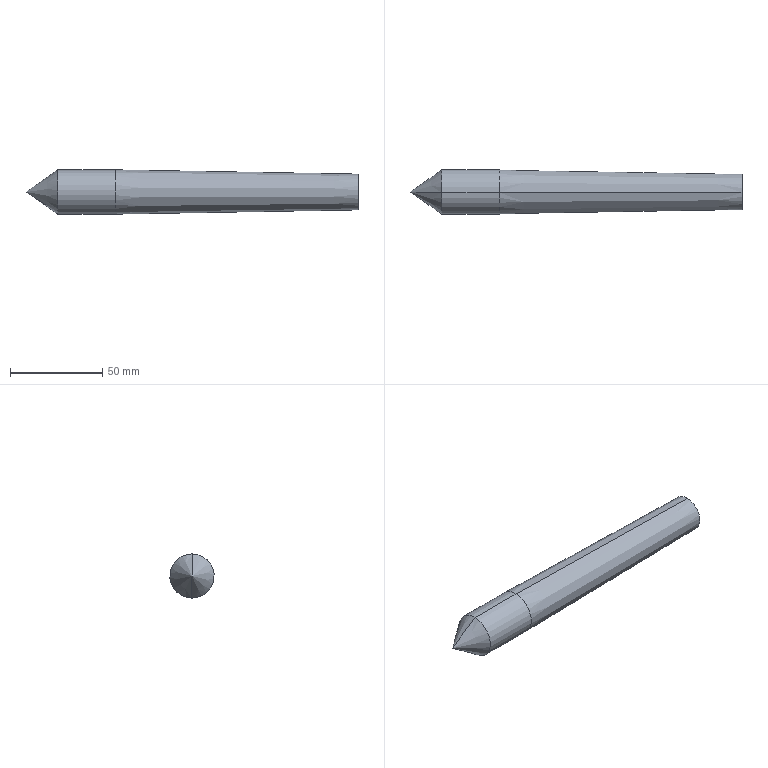Component | SolidWorks | LiveCenter-2 | 1 solid | 7 faces | box 180 x 24 x 24 mm | volume 65614 mm3 | cone 4 | cylinder 2 | plane 1 | commonest cylinder face diameters 24 x2
build123d program:
from build123d import *


with BuildPart() as part:
    # Sketch1 → Revolve1 (revolve)
    with BuildSketch(Plane.XY, mode=Mode.PRIVATE) as revolve1_sk:
        Polygon((-48.539, 12), (-31.401, 24), (0, 24), (131.461, 21.705), (131.461, 12), (5.947, 12), align=None)
    revolve(revolve1_sk.sketch.rotate(Axis((-48.539, 12, 0), (1, 0, 0)), 90), axis=Axis((-48.539, 12, 0), (1, 0, 0)))


solid = part.part

# Placed as in the assembly
solid = solid.moved(Location((-139.78, 138, -15), (0, 0, 0)))
STEP:
#1=COLOUR_RGB('',0.7922,0.8196,0.9333);
#2=FILL_AREA_STYLE_COLOUR('',#1);
#3=FILL_AREA_STYLE('',(#2));
#4=SURFACE_STYLE_FILL_AREA(#3);
#5=SURFACE_SIDE_STYLE('',(#4));
#6=SURFACE_STYLE_USAGE(.BOTH.,#5);
#7=PRESENTATION_STYLE_ASSIGNMENT((#6));
#8=CARTESIAN_POINT('',(-0.3275,5.896,-0.2086));
#9=VERTEX_POINT('',#8);
#10=CARTESIAN_POINT('',(-0.3275,5.915,-0.9725));
#11=VERTEX_POINT('',#10);
#12=CARTESIAN_POINT('',(-0.3275,5.906,-0.5906));
#13=DIRECTION('',(-1.,0.,0.));
#14=DIRECTION('',(0.,-0.02554,0.9997));
#15=AXIS2_PLACEMENT_3D('',#12,#13,#14);
#16=CIRCLE('',#15,0.3821);
#17=EDGE_CURVE('',#9,#11,#16,.T.);
#18=ORIENTED_EDGE('',*,*,#17,.T.);
#19=CARTESIAN_POINT('',(-5.503,5.918,-1.063));
#20=VERTEX_POINT('',#19);
#21=CARTESIAN_POINT('',(-0.3275,5.915,-0.9725));
#22=DIRECTION('',(-0.9998,0.0004457,-0.01745));
#23=VECTOR('',#22,39.37);
#24=LINE('',#21,#23);
#25=EDGE_CURVE('',#11,#20,#24,.T.);
#26=ORIENTED_EDGE('',*,*,#25,.T.);
#27=CARTESIAN_POINT('',(-5.503,5.893,-0.1183));
#28=VERTEX_POINT('',#27);
#29=CARTESIAN_POINT('',(-5.503,5.906,-0.5906));
#30=DIRECTION('',(-1.,0.,0.));
#31=DIRECTION('',(0.,-0.02554,0.9997));
#32=AXIS2_PLACEMENT_3D('',#29,#30,#31);
#33=CIRCLE('',#32,0.4724);
#34=EDGE_CURVE('',#28,#20,#33,.T.);
#35=ORIENTED_EDGE('',*,*,#34,.F.);
#36=CARTESIAN_POINT('',(-0.3275,5.896,-0.2086));
#37=DIRECTION('',(-0.9998,-0.0004457,0.01745));
#38=VECTOR('',#37,39.37);
#39=LINE('',#36,#38);
#40=EDGE_CURVE('',#9,#28,#39,.T.);
#41=ORIENTED_EDGE('',*,*,#40,.F.);
#42=EDGE_LOOP('',(#18,#26,#35,#41));
#43=FACE_OUTER_BOUND('',#42,.T.);
#44=CARTESIAN_POINT('',(-0.3275,5.906,-0.5906));
#45=DIRECTION('',(-1.,0.,0.));
#46=DIRECTION('',(0.,-0.02554,0.9997));
#47=AXIS2_PLACEMENT_3D('',#44,#45,#46);
#48=CONICAL_SURFACE('',#47,0.3821,0.01745);
#49=ADVANCED_FACE('',(#43),#48,.T.);
#50=ORIENTED_EDGE('',*,*,#34,.T.);
#51=CARTESIAN_POINT('',(-6.739,5.918,-1.063));
#52=VERTEX_POINT('',#51);
#53=CARTESIAN_POINT('',(-7.414,5.918,-1.063));
#54=DIRECTION('',(-1.,0.,0.));
#55=VECTOR('',#54,39.37);
#56=LINE('',#53,#55);
#57=EDGE_CURVE('',#20,#52,#56,.T.);
#58=ORIENTED_EDGE('',*,*,#57,.T.);
#59=CARTESIAN_POINT('',(-6.739,5.893,-0.1183));
#60=VERTEX_POINT('',#59);
#61=CARTESIAN_POINT('',(-6.739,5.906,-0.5906));
#62=DIRECTION('',(-1.,0.,0.));
#63=DIRECTION('',(0.,-0.02554,0.9997));
#64=AXIS2_PLACEMENT_3D('',#61,#62,#63);
#65=CIRCLE('',#64,0.4724);
#66=EDGE_CURVE('',#60,#52,#65,.T.);
#67=ORIENTED_EDGE('',*,*,#66,.F.);
#68=CARTESIAN_POINT('',(-7.414,5.893,-0.1183));
#69=DIRECTION('',(-1.,0.,0.));
#70=VECTOR('',#69,39.37);
#71=LINE('',#68,#70);
#72=EDGE_CURVE('',#28,#60,#71,.T.);
#73=ORIENTED_EDGE('',*,*,#72,.F.);
#74=EDGE_LOOP('',(#50,#58,#67,#73));
#75=FACE_OUTER_BOUND('',#74,.T.);
#76=CARTESIAN_POINT('',(-7.414,5.906,-0.5906));
#77=DIRECTION('',(-1.,0.,0.));
#78=DIRECTION('',(0.,-0.02554,0.9997));
#79=AXIS2_PLACEMENT_3D('',#76,#77,#78);
#80=CYLINDRICAL_SURFACE('',#79,0.4724);
#81=ADVANCED_FACE('',(#75),#80,.T.);
#82=CARTESIAN_POINT('',(-7.414,5.906,-0.5906));
#83=VERTEX_POINT('',#82);
#84=CARTESIAN_POINT('',(-6.739,5.918,-1.063));
#85=DIRECTION('',(0.8192,0.01465,-0.5734));
#86=VECTOR('',#85,39.37);
#87=LINE('',#84,#86);
#88=EDGE_CURVE('',#83,#52,#87,.T.);
#89=ORIENTED_EDGE('',*,*,#88,.F.);
#90=CARTESIAN_POINT('',(-6.739,5.893,-0.1183));
#91=DIRECTION('',(0.8192,-0.01465,0.5734));
#92=VECTOR('',#91,39.37);
#93=LINE('',#90,#92);
#94=EDGE_CURVE('',#83,#60,#93,.T.);
#95=ORIENTED_EDGE('',*,*,#94,.T.);
#96=ORIENTED_EDGE('',*,*,#66,.T.);
#97=EDGE_LOOP('',(#89,#95,#96));
#98=FACE_OUTER_BOUND('',#97,.T.);
#99=CARTESIAN_POINT('',(-6.739,5.906,-0.5906));
#100=DIRECTION('',(1.,0.,0.));
#101=DIRECTION('',(0.,0.02554,-0.9997));
#102=AXIS2_PLACEMENT_3D('',#99,#100,#101);
#103=CONICAL_SURFACE('',#102,0.4724,0.6109);
#104=ADVANCED_FACE('',(#98),#103,.T.);
#105=ORIENTED_EDGE('',*,*,#94,.F.);
#106=ORIENTED_EDGE('',*,*,#88,.T.);
#107=CARTESIAN_POINT('',(-6.739,5.906,-0.5906));
#108=DIRECTION('',(-1.,0.,0.));
#109=DIRECTION('',(0.,-0.02554,0.9997));
#110=AXIS2_PLACEMENT_3D('',#107,#108,#109);
#111=CIRCLE('',#110,0.4724);
#112=EDGE_CURVE('',#52,#60,#111,.T.);
#113=ORIENTED_EDGE('',*,*,#112,.T.);
#114=EDGE_LOOP('',(#105,#106,#113));
#115=FACE_OUTER_BOUND('',#114,.T.);
#116=CARTESIAN_POINT('',(-6.739,5.906,-0.5906));
#117=DIRECTION('',(1.,0.,0.));
#118=DIRECTION('',(0.,0.02554,-0.9997));
#119=AXIS2_PLACEMENT_3D('',#116,#117,#118);
#120=CONICAL_SURFACE('',#119,0.4724,0.6109);
#121=ADVANCED_FACE('',(#115),#120,.T.);
#122=ORIENTED_EDGE('',*,*,#57,.F.);
#123=CARTESIAN_POINT('',(-5.503,5.906,-0.5906));
#124=DIRECTION('',(-1.,0.,0.));
#125=DIRECTION('',(0.,-0.02554,0.9997));
#126=AXIS2_PLACEMENT_3D('',#123,#124,#125);
#127=CIRCLE('',#126,0.4724);
#128=EDGE_CURVE('',#20,#28,#127,.T.);
#129=ORIENTED_EDGE('',*,*,#128,.T.);
#130=ORIENTED_EDGE('',*,*,#72,.T.);
#131=ORIENTED_EDGE('',*,*,#112,.F.);
#132=EDGE_LOOP('',(#122,#129,#130,#131));
#133=FACE_OUTER_BOUND('',#132,.T.);
#134=CARTESIAN_POINT('',(-7.414,5.906,-0.5906));
#135=DIRECTION('',(-1.,0.,0.));
#136=DIRECTION('',(0.,-0.02554,0.9997));
#137=AXIS2_PLACEMENT_3D('',#134,#135,#136);
#138=CYLINDRICAL_SURFACE('',#137,0.4724);
#139=ADVANCED_FACE('',(#133),#138,.T.);
#140=ORIENTED_EDGE('',*,*,#25,.F.);
#141=CARTESIAN_POINT('',(-0.3275,5.906,-0.5906));
#142=DIRECTION('',(-1.,0.,0.));
#143=DIRECTION('',(0.,-0.02554,0.9997));
#144=AXIS2_PLACEMENT_3D('',#141,#142,#143);
#145=CIRCLE('',#144,0.3821);
#146=EDGE_CURVE('',#11,#9,#145,.T.);
#147=ORIENTED_EDGE('',*,*,#146,.T.);
#148=ORIENTED_EDGE('',*,*,#40,.T.);
#149=ORIENTED_EDGE('',*,*,#128,.F.);
#150=EDGE_LOOP('',(#140,#147,#148,#149));
#151=FACE_OUTER_BOUND('',#150,.T.);
#152=CARTESIAN_POINT('',(-0.3275,5.906,-0.5906));
#153=DIRECTION('',(-1.,0.,0.));
#154=DIRECTION('',(0.,-0.02554,0.9997));
#155=AXIS2_PLACEMENT_3D('',#152,#153,#154);
#156=CONICAL_SURFACE('',#155,0.3821,0.01745);
#157=ADVANCED_FACE('',(#151),#156,.T.);
#158=ORIENTED_EDGE('',*,*,#17,.F.);
#159=ORIENTED_EDGE('',*,*,#146,.F.);
#160=EDGE_LOOP('',(#158,#159));
#161=FACE_OUTER_BOUND('',#160,.T.);
#162=CARTESIAN_POINT('',(-0.3275,6.287,-0.5808));
#163=DIRECTION('',(-1.,0.,0.));
#164=DIRECTION('',(0.,-0.02554,0.9997));
#165=AXIS2_PLACEMENT_3D('',#162,#163,#164);
#166=PLANE('',#165);
#167=ADVANCED_FACE('',(#161),#166,.F.);
#168=CLOSED_SHELL('',(#49,#81,#104,#121,#139,#157,#167));
#169=MANIFOLD_SOLID_BREP('',#168);
#170=STYLED_ITEM('',(#7),#169);
#171=(LENGTH_UNIT()NAMED_UNIT(*)SI_UNIT($,.METRE.));
#172=LENGTH_MEASURE_WITH_UNIT(LENGTH_MEASURE(0.0254),#171);
#173=DIMENSIONAL_EXPONENTS(1.,0.,0.,0.,0.,0.,0.);
#174=(CONVERSION_BASED_UNIT('',#172)LENGTH_UNIT()NAMED_UNIT(#173));
#175=UNCERTAINTY_MEASURE_WITH_UNIT(LENGTH_MEASURE(0.00001),#174,'','');
#176=(NAMED_UNIT(*)PLANE_ANGLE_UNIT()SI_UNIT($,.RADIAN.));
#177=(NAMED_UNIT(*)SI_UNIT($,.STERADIAN.)SOLID_ANGLE_UNIT());
#178=(GEOMETRIC_REPRESENTATION_CONTEXT(3)GLOBAL_UNCERTAINTY_ASSIGNED_CONTEXT((#175))GLOBAL_UNIT_ASSIGNED_CONTEXT((#174,#176,#177))REPRESENTATION_CONTEXT('',''));
#179=MECHANICAL_DESIGN_GEOMETRIC_PRESENTATION_REPRESENTATION('',(#170),#178);
#180=PRESENTATION_LAYER_ASSIGNMENT('','',(#170));
#181=CARTESIAN_POINT('',(0.,0.,0.));
#182=DIRECTION('',(0.,0.,1.));
#183=DIRECTION('',(1.,0.,0.));
#184=AXIS2_PLACEMENT_3D('',#181,#182,#183);
#185=(LENGTH_UNIT()NAMED_UNIT(*)SI_UNIT($,.METRE.));
#186=LENGTH_MEASURE_WITH_UNIT(LENGTH_MEASURE(0.0254),#185);
#187=DIMENSIONAL_EXPONENTS(1.,0.,0.,0.,0.,0.,0.);
#188=(CONVERSION_BASED_UNIT('',#186)LENGTH_UNIT()NAMED_UNIT(#187));
#189=UNCERTAINTY_MEASURE_WITH_UNIT(LENGTH_MEASURE(0.00001),#188,'','');
#190=(NAMED_UNIT(*)PLANE_ANGLE_UNIT()SI_UNIT($,.RADIAN.));
#191=(NAMED_UNIT(*)SI_UNIT($,.STERADIAN.)SOLID_ANGLE_UNIT());
#192=(GEOMETRIC_REPRESENTATION_CONTEXT(3)GLOBAL_UNCERTAINTY_ASSIGNED_CONTEXT((#189))GLOBAL_UNIT_ASSIGNED_CONTEXT((#188,#190,#191))REPRESENTATION_CONTEXT('',''));
#193=ADVANCED_BREP_SHAPE_REPRESENTATION('',(#169,#184),#192);